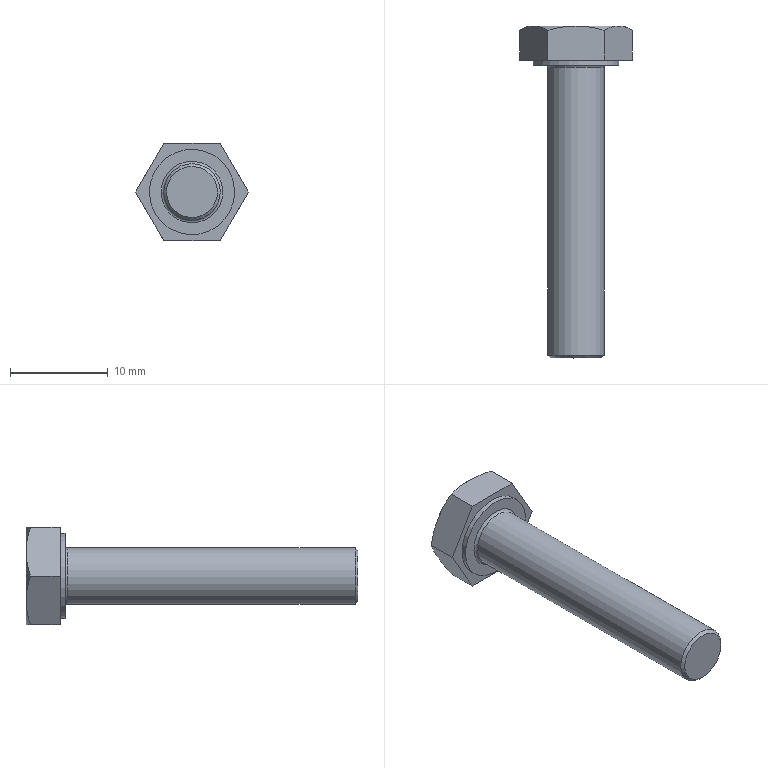Component | NX | BOLT_M6X30_4 | 1 solid | 20 faces | volume 1123 mm3 | plane 10 | cone 7 | cylinder 2 | torus 1 | commonest cylinder face diameters 8.74 x1 5.795 x1